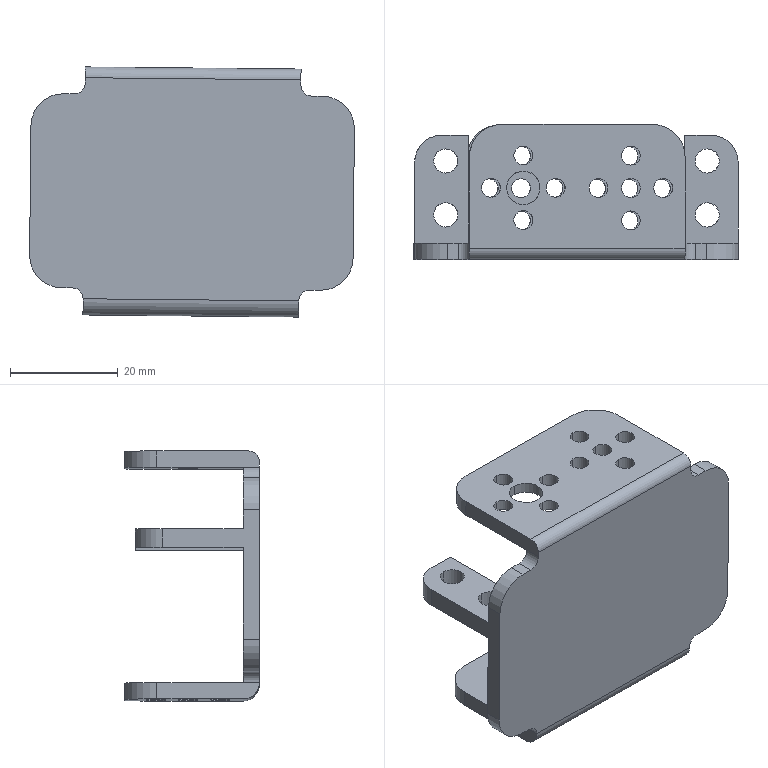Component | SolidWorks | Bracket2-1 | 1 solid | 95 faces | box 60.23 x 25 x 46.39 mm | volume 13092 mm3 | cylinder 68 | plane 27 | commonest cylinder face diameters 3.5 x38 4.5 x8 12 x8 4 x5 12.8 x4 6.2 x2 10 x2 6 x1 | material 45
build123d program:
from build123d import *

# Parameters (mm, degrees)
SKETCH1_2_W                   = 60
SKETCH1_2_H                   = 36
BOSS_EXTRUDE1_DEPTH           = 3
BOSS_EXTRUDE2_DEPTH           = 20
FILLET2_R                     = 3
FILLET3_R                     = 2
FILLET4_R                     = 2
FILLET5_R                     = 2
FILLET6_R                     = 6
FILLET7_R                     = 6
SKETCH4_R                     = 1.75
CUT_EXTRUDE1_DEPTH            = 64.239
SKETCH6_W                     = 10.083
SKETCH6_H                     = 3.5
SKETCH6_W_2                   = 10
BOSS_EXTRUDE3_DEPTH           = 20
FILLET8_R                     = 5
SKETCH7_R                     = 2.25
CUT_EXTRUDE2_DEPTH            = 54.623
SKETCH8_R                     = 3.1
CUT_EXTRUDE3_DEPTH            = 20
SKETCH9_R                     = 1.75
CUT_EXTRUDE4_DEPTH            = 64.239
SKETCH10_R                    = 1.75
CUT_EXTRUDE5_DEPTH            = 20
SKETCH1_W                     = 0.5
SKETCH1_H                     = 20.6
RELIEF_FLANGETABCASEEND_DEPTH = 3.6
SKETCH2_R                     = 6.4
COUNTERBORE_SERVOBOSS_DEPTH   = 1


with BuildPart() as part:
    # Sketch1_2 → Boss-Extrude1 (new body)
    with BuildSketch(Plane.XY):
        with Locations((5.47, 1.846)):
            Rectangle(SKETCH1_2_W, SKETCH1_2_H)
    extrude(amount=BOSS_EXTRUDE1_DEPTH)

    # Sketch3 → Boss-Extrude2 (add, symmetric)
    with BuildSketch(Plane(origin=(5.47, 0, 0), x_dir=(0, 0, -1), z_dir=(1, 0, 0))):
        Polygon((0, 22.87), (0, 24.846), (-25, 24.846), (-25, 21.846), (-3, 21.846), (-3, 19.846), (0, 19.846), align=None)
    boss_extrude2 = extrude(amount=BOSS_EXTRUDE2_DEPTH, both=True)

    # Fillet2
    fillet2_edges = [part.edges().sort_by_distance(p)[0] for p in [
        (5.47, 24.846, 0),
    ]]
    fillet(fillet2_edges, radius=FILLET2_R)

    # Fillet3
    fillet3_edges = [part.edges().sort_by_distance(p)[0] for p in [
        (-14.53, 19.846, 1.5),
        (25.47, 19.846, 1.5),
    ]]
    fillet(fillet3_edges, radius=FILLET3_R)

    # Mirror2: Boss-Extrude2 across plane
    add(boss_extrude2.mirror(Plane(origin=(0, 1.846, 0), x_dir=(0, 0, 1), z_dir=(0, -1, 0))))

    # Fillet4
    fillet4_edges = [part.edges().sort_by_distance(p)[0] for p in [
        (25.47, -16.154, 1.5),
        (-14.53, -16.154, 1.5),
    ]]
    fillet(fillet4_edges, radius=FILLET4_R)

    # Fillet5
    fillet5_edges = [part.edges().sort_by_distance(p)[0] for p in [
        (5.47, -21.154, 0),
    ]]
    fillet(fillet5_edges, radius=FILLET5_R)

    # Fillet6
    fillet6_edges = [part.edges().sort_by_distance(p)[0] for p in [
        (-24.53, -16.154, 1.5),
        (-24.53, 19.846, 1.5),
        (35.47, -16.154, 1.5),
        (35.47, 19.846, 1.5),
    ]]
    fillet(fillet6_edges, radius=FILLET6_R)

    # Fillet7
    fillet7_edges = [part.edges().sort_by_distance(p)[0] for p in [
        (-14.53, 23.346, 25),
        (25.47, 23.346, 25),
        (25.47, -19.654, 25),
        (-14.53, -19.654, 25),
    ]]
    fillet(fillet7_edges, radius=FILLET7_R)

    # Sketch4 → Cut-Extrude1 (cut, through all)
    with BuildSketch(Plane(origin=(0, 24.846, 0), x_dir=(1, 0, 0), z_dir=(0, 1, 0))):
        with Locations(Location((15.424, -19.2, 0), (0, 0, 270))):
            Circle(SKETCH4_R)
        with Locations(Location((9.424, -13.2, 0), (0, 0, 270))):
            Circle(SKETCH4_R)
        with Locations(Location((15.424, -7.2, 0), (0, 0, 270))):
            Circle(SKETCH4_R)
        with Locations(Location((21.424, -13.2, 0), (0, 0, 270))):
            Circle(SKETCH4_R)
        with Locations(Location((15.424, -13.2, 0), (0, 0, 270))):
            Circle(SKETCH4_R)
    extrude(amount=-CUT_EXTRUDE1_DEPTH, mode=Mode.SUBTRACT)

    # Sketch6 → Boss-Extrude3 (add)
    with BuildSketch(Plane.XY.offset(3)):
        with Locations((30.429, -4.904)):
            Rectangle(SKETCH6_W, SKETCH6_H)
        with Locations((-19.53, -4.904)):
            Rectangle(SKETCH6_W_2, SKETCH6_H)
    extrude(amount=BOSS_EXTRUDE3_DEPTH)

    # Fillet8
    fillet8_edges = [part.edges().sort_by_distance(p)[0] for p in [
        (35.47, -4.904, 23),
        (-24.53, -4.904, 23),
    ]]
    fillet(fillet8_edges, radius=FILLET8_R)

    # Sketch7 → Cut-Extrude2 (cut, through all)
    with BuildSketch(Plane.XZ.offset(6.654)):
        with Locations(Location((29.72, 18.243, 0), (0, 0, 270))):
            Circle(SKETCH7_R)
        with Locations(Location((29.72, 8.243, 0), (0, 0, 270))):
            Circle(SKETCH7_R)
        with Locations(Location((-18.78, 18.243, 0), (0, 0, 270))):
            Circle(SKETCH7_R)
        with Locations(Location((-18.78, 8.243, 0), (0, 0, 270))):
            Circle(SKETCH7_R)
    extrude(amount=-CUT_EXTRUDE2_DEPTH, mode=Mode.SUBTRACT)

    # Sketch8 → Cut-Extrude3 (cut)
    with BuildSketch(Plane.XZ.offset(21.154)):
        with Locations(Location((-4.53, 13.243, 0), (0, 0, 270))):
            Circle(SKETCH8_R)
    extrude(amount=-CUT_EXTRUDE3_DEPTH, mode=Mode.SUBTRACT)

    # Sketch9 → Cut-Extrude4 (cut, through all)
    with BuildSketch(Plane.XZ.offset(21.154)):
        with Locations(Location((-4.53, 19.243, 0), (0, 0, 270))):
            Circle(SKETCH9_R)
        with Locations(Location((1.47, 13.243, 0), (0, 0, 270))):
            Circle(SKETCH9_R)
        with Locations(Location((-4.53, 7.243, 0), (0, 0, 270))):
            Circle(SKETCH9_R)
        with Locations(Location((-10.53, 13.243, 0), (0, 0, 270))):
            Circle(SKETCH9_R)
    extrude(amount=-CUT_EXTRUDE4_DEPTH, mode=Mode.SUBTRACT)

    # Sketch10 → Cut-Extrude5 (cut)
    with BuildSketch(Plane(origin=(0, 24.846, 0), x_dir=(1, 0, 0), z_dir=(0, 1, 0))):
        with Locations(Location((-4.53, -13.243, 0), (0, 0, 270))):
            Circle(SKETCH10_R)
    extrude(amount=-CUT_EXTRUDE5_DEPTH, mode=Mode.SUBTRACT)

    # Sketch1 → Relief-FlangeTabCaseEnd (cut)
    with BuildSketch(Plane.XZ.offset(6.654)):
        with Locations((25.32, 13.3)):
            Rectangle(SKETCH1_W, SKETCH1_H)
    extrude(amount=-RELIEF_FLANGETABCASEEND_DEPTH, mode=Mode.SUBTRACT)

    # Sketch2 → Counterbore-ServoBoss (cut)
    with BuildSketch(Plane(origin=(0, -18.154, 0), x_dir=(1, 0, 0), z_dir=(0, 1, 0))):
        with Locations((-4.53, -13.24)):
            Circle(SKETCH2_R)
    extrude(amount=-COUNTERBORE_SERVOBOSS_DEPTH, mode=Mode.SUBTRACT)


solid = part.part

# Placed as in the assembly
solid = solid.moved(Location((0, 17.25, 0), (-90, 0, 0.5611)))